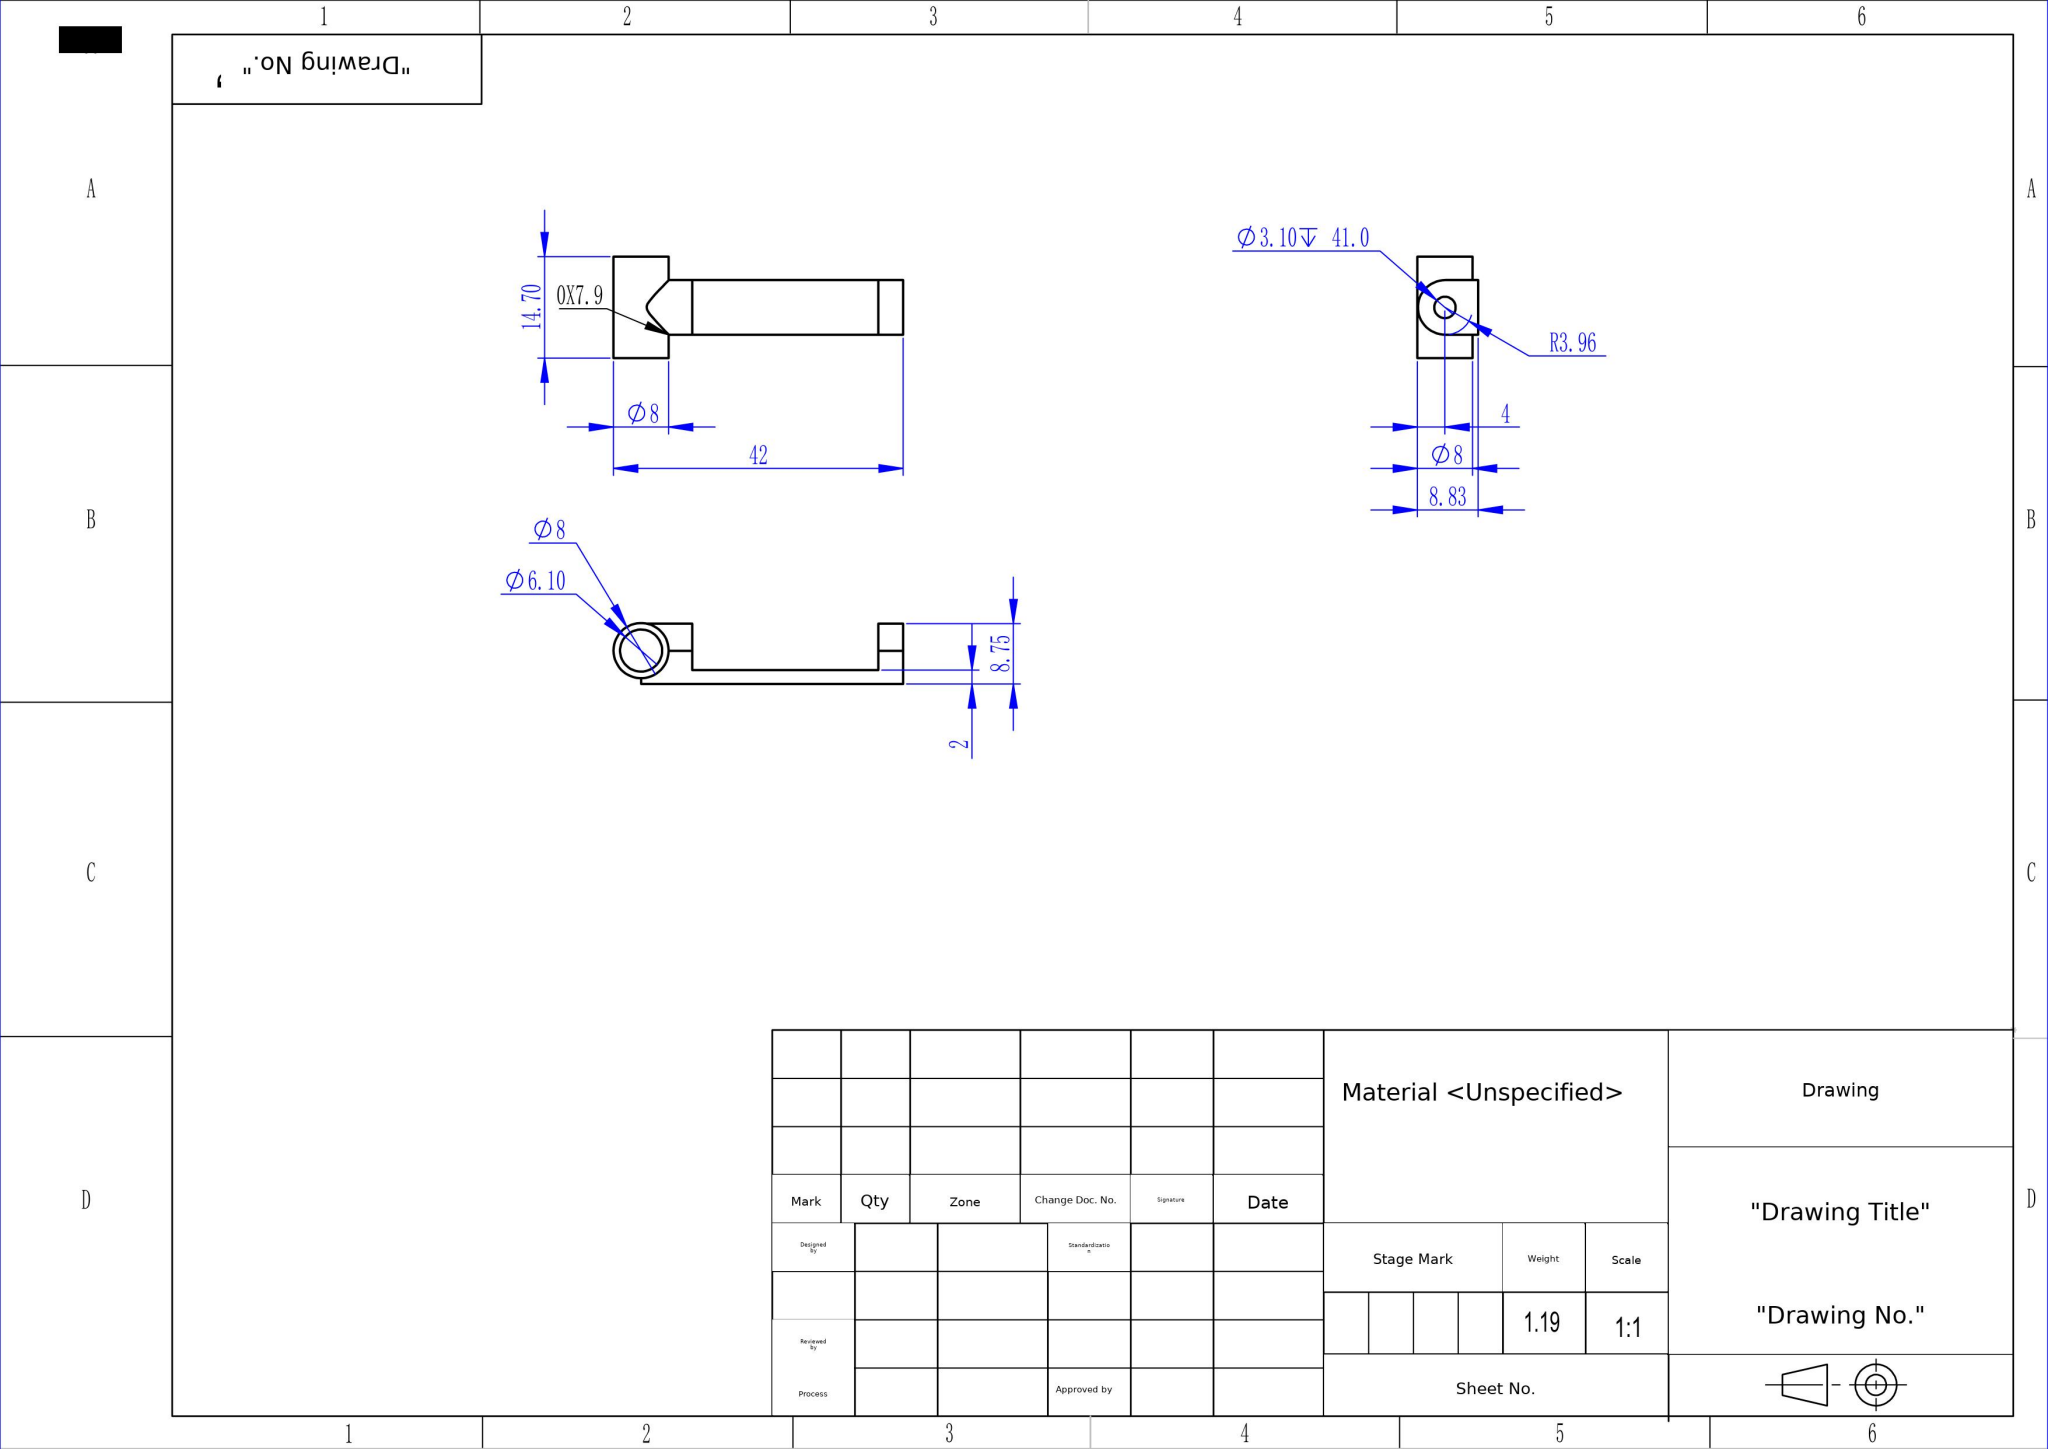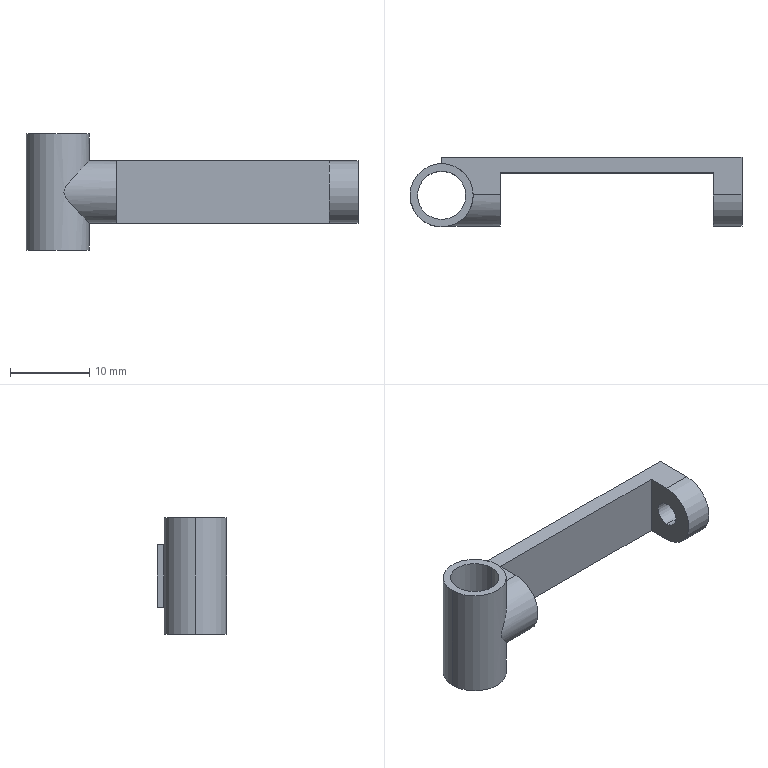Part | SolidWorks | mm | 1 solid | 21 faces | box 42 x 8.83 x 14.7 mm | volume 1194 mm3 | plane 11 | cylinder 10 | commonest cylinder face diameters 3.1 x4 6.1 x2 8 x2 7.923 x2
build123d program:
from build123d import *

# Parameters (mm, degrees)
SKETCH1_R           = 4
SKETCH1_R_2         = 3.05
BOSS_EXTRUDE1_DEPTH = 14.7
BOSS_EXTRUDE2_DEPTH = 38
CUT_EXTRUDE1_START  = -2
SKETCH3_W           = 26.966
SKETCH3_H           = 7.923
CUT_EXTRUDE1_DEPTH  = 30
CUT_EXTRUDE2_START  = -3
SKETCH4_R           = 1.55
CUT_EXTRUDE2_DEPTH  = 41
SKETCH5_R           = 3.05
CUT_EXTRUDE3_DEPTH  = 17


with BuildPart() as part:
    # Sketch1 → Boss-Extrude1 (new body)
    with BuildSketch(Plane.XY):
        Circle(SKETCH1_R)
        Circle(SKETCH1_R_2, mode=Mode.SUBTRACT)
    extrude(amount=BOSS_EXTRUDE1_DEPTH)

    # Sketch2 → Boss-Extrude2 (add)
    with BuildSketch(Plane(origin=(0, 0, 0), x_dir=(0, 0, -1), z_dir=(1, 0, 0))):
        with BuildLine():
            Line((-3.389, 4.83), (-11.311, 4.83))
            Line((-11.311, 4.83), (-11.311, 0.04196))
            ThreePointArc((-11.311, 0.04196), (-7.35, -3.919), (-3.389, 0.04196))
            Line((-3.389, 0.04196), (-3.389, 4.83))
        make_face()
    extrude(amount=BOSS_EXTRUDE2_DEPTH)

    # Sketch3 → Cut-Extrude1 (cut)
    with BuildSketch(Plane(origin=(0, 4.83, 0), x_dir=(1, 0, 0), z_dir=(0, 1, 0)).offset(CUT_EXTRUDE1_START)):
        with Locations((20.909, -7.35)):
            Rectangle(SKETCH3_W, SKETCH3_H)
    extrude(amount=-CUT_EXTRUDE1_DEPTH, mode=Mode.SUBTRACT)

    # Sketch4 → Cut-Extrude2 (cut)
    with BuildSketch(Plane(origin=(7.426, 0, 0), x_dir=(0, 0, -1), z_dir=(1, 0, 0)).offset(CUT_EXTRUDE2_START)):
        with Locations(Location((-7.35, 0, 0), (0, 0, 180))):
            Circle(SKETCH4_R)
    extrude(amount=CUT_EXTRUDE2_DEPTH, mode=Mode.SUBTRACT)

    # Sketch5 → Cut-Extrude3 (cut)
    with BuildSketch(Plane(origin=(0, 0, 0), x_dir=(-1, 0, 0), z_dir=(0, 0, -1))):
        with Locations(Location((0, 0, 0), (0, 0, 180))):
            Circle(SKETCH5_R)
    extrude(amount=-CUT_EXTRUDE3_DEPTH, mode=Mode.SUBTRACT)


solid = part.part
STEP:
#1=CARTESIAN_POINT('',(38.,0.,5.8));
#2=VERTEX_POINT('',#1);
#3=CARTESIAN_POINT('',(38.,0.,8.9));
#4=VERTEX_POINT('',#3);
#5=CARTESIAN_POINT('',(38.,0.,7.35));
#6=DIRECTION('',(-1.,0.,0.));
#7=DIRECTION('',(0.,0.,-1.));
#8=AXIS2_PLACEMENT_3D('',#5,#6,#7);
#9=CIRCLE('',#8,1.55);
#10=EDGE_CURVE('',#2,#4,#9,.T.);
#11=ORIENTED_EDGE('',*,*,#10,.F.);
#12=CARTESIAN_POINT('',(34.392,0.,5.8));
#13=VERTEX_POINT('',#12);
#14=CARTESIAN_POINT('',(45.426,0.,5.8));
#15=DIRECTION('',(-1.,0.,0.));
#16=VECTOR('',#15,1000.);
#17=LINE('',#14,#16);
#18=EDGE_CURVE('',#2,#13,#17,.T.);
#19=ORIENTED_EDGE('',*,*,#18,.T.);
#20=CARTESIAN_POINT('',(34.392,0.,8.9));
#21=VERTEX_POINT('',#20);
#22=CARTESIAN_POINT('',(34.392,0.,7.35));
#23=DIRECTION('',(-1.,0.,0.));
#24=DIRECTION('',(0.,0.,-1.));
#25=AXIS2_PLACEMENT_3D('',#22,#23,#24);
#26=CIRCLE('',#25,1.55);
#27=EDGE_CURVE('',#13,#21,#26,.T.);
#28=ORIENTED_EDGE('',*,*,#27,.T.);
#29=CARTESIAN_POINT('',(45.426,0.,8.9));
#30=DIRECTION('',(-1.,0.,0.));
#31=VECTOR('',#30,1000.);
#32=LINE('',#29,#31);
#33=EDGE_CURVE('',#4,#21,#32,.T.);
#34=ORIENTED_EDGE('',*,*,#33,.F.);
#35=EDGE_LOOP('',(#11,#19,#28,#34));
#36=FACE_OUTER_BOUND('',#35,.T.);
#37=CARTESIAN_POINT('',(45.426,0.,7.35));
#38=DIRECTION('',(-1.,0.,0.));
#39=DIRECTION('',(0.,0.,1.));
#40=AXIS2_PLACEMENT_3D('',#37,#38,#39);
#41=CYLINDRICAL_SURFACE('',#40,1.55);
#42=ADVANCED_FACE('',(#36),#41,.F.);
#43=CARTESIAN_POINT('',(7.426,0.,8.9));
#44=VERTEX_POINT('',#43);
#45=CARTESIAN_POINT('',(7.426,0.,5.8));
#46=VERTEX_POINT('',#45);
#47=CARTESIAN_POINT('',(7.426,0.,7.35));
#48=DIRECTION('',(1.,0.,0.));
#49=DIRECTION('',(0.,0.,1.));
#50=AXIS2_PLACEMENT_3D('',#47,#48,#49);
#51=CIRCLE('',#50,1.55);
#52=EDGE_CURVE('',#44,#46,#51,.T.);
#53=ORIENTED_EDGE('',*,*,#52,.T.);
#54=CARTESIAN_POINT('',(4.426,0.,5.8));
#55=VERTEX_POINT('',#54);
#56=CARTESIAN_POINT('',(45.426,0.,5.8));
#57=DIRECTION('',(-1.,0.,0.));
#58=VECTOR('',#57,1000.);
#59=LINE('',#56,#58);
#60=EDGE_CURVE('',#46,#55,#59,.T.);
#61=ORIENTED_EDGE('',*,*,#60,.T.);
#62=CARTESIAN_POINT('',(4.426,0.,8.9));
#63=VERTEX_POINT('',#62);
#64=CARTESIAN_POINT('',(4.426,0.,7.35));
#65=DIRECTION('',(1.,0.,0.));
#66=DIRECTION('',(0.,0.,-1.));
#67=AXIS2_PLACEMENT_3D('',#64,#65,#66);
#68=CIRCLE('',#67,1.55);
#69=EDGE_CURVE('',#63,#55,#68,.T.);
#70=ORIENTED_EDGE('',*,*,#69,.F.);
#71=CARTESIAN_POINT('',(45.426,0.,8.9));
#72=DIRECTION('',(-1.,0.,0.));
#73=VECTOR('',#72,1000.);
#74=LINE('',#71,#73);
#75=EDGE_CURVE('',#44,#63,#74,.T.);
#76=ORIENTED_EDGE('',*,*,#75,.F.);
#77=EDGE_LOOP('',(#53,#61,#70,#76));
#78=FACE_OUTER_BOUND('',#77,.T.);
#79=CARTESIAN_POINT('',(45.426,0.,7.35));
#80=DIRECTION('',(-1.,0.,0.));
#81=DIRECTION('',(0.,0.,1.));
#82=AXIS2_PLACEMENT_3D('',#79,#80,#81);
#83=CYLINDRICAL_SURFACE('',#82,1.55);
#84=ADVANCED_FACE('',(#78),#83,.F.);
#85=CARTESIAN_POINT('',(-3.05,0.,14.7));
#86=VERTEX_POINT('',#85);
#87=CARTESIAN_POINT('',(3.05,0.,14.7));
#88=VERTEX_POINT('',#87);
#89=CARTESIAN_POINT('',(0.,0.,14.7));
#90=DIRECTION('',(0.,0.,1.));
#91=DIRECTION('',(1.,0.,0.));
#92=AXIS2_PLACEMENT_3D('',#89,#90,#91);
#93=CIRCLE('',#92,3.05);
#94=EDGE_CURVE('',#86,#88,#93,.T.);
#95=ORIENTED_EDGE('',*,*,#94,.T.);
#96=CARTESIAN_POINT('',(3.05,0.,0.));
#97=VERTEX_POINT('',#96);
#98=CARTESIAN_POINT('',(3.05,0.,14.7));
#99=DIRECTION('',(0.,0.,-1.));
#100=VECTOR('',#99,1000.);
#101=LINE('',#98,#100);
#102=EDGE_CURVE('',#88,#97,#101,.T.);
#103=ORIENTED_EDGE('',*,*,#102,.T.);
#104=CARTESIAN_POINT('',(-3.05,0.,0.));
#105=VERTEX_POINT('',#104);
#106=CARTESIAN_POINT('',(0.,0.,0.));
#107=DIRECTION('',(0.,0.,1.));
#108=DIRECTION('',(1.,0.,0.));
#109=AXIS2_PLACEMENT_3D('',#106,#107,#108);
#110=CIRCLE('',#109,3.05);
#111=EDGE_CURVE('',#105,#97,#110,.T.);
#112=ORIENTED_EDGE('',*,*,#111,.F.);
#113=CARTESIAN_POINT('',(-3.05,0.,14.7));
#114=DIRECTION('',(0.,0.,-1.));
#115=VECTOR('',#114,1000.);
#116=LINE('',#113,#115);
#117=EDGE_CURVE('',#86,#105,#116,.T.);
#118=ORIENTED_EDGE('',*,*,#117,.F.);
#119=EDGE_LOOP('',(#95,#103,#112,#118));
#120=FACE_OUTER_BOUND('',#119,.T.);
#121=CARTESIAN_POINT('',(0.,0.,14.7));
#122=DIRECTION('',(0.,0.,-1.));
#123=DIRECTION('',(-1.,0.,0.));
#124=AXIS2_PLACEMENT_3D('',#121,#122,#123);
#125=CYLINDRICAL_SURFACE('',#124,3.05);
#126=ADVANCED_FACE('',(#120),#125,.F.);
#127=CARTESIAN_POINT('',(4.,0.,14.7));
#128=VERTEX_POINT('',#127);
#129=CARTESIAN_POINT('',(-4.,0.,14.7));
#130=VERTEX_POINT('',#129);
#131=CARTESIAN_POINT('',(0.,0.,14.7));
#132=DIRECTION('',(0.,0.,1.));
#133=DIRECTION('',(1.,0.,0.));
#134=AXIS2_PLACEMENT_3D('',#131,#132,#133);
#135=CIRCLE('',#134,4.);
#136=EDGE_CURVE('',#128,#130,#135,.T.);
#137=ORIENTED_EDGE('',*,*,#136,.F.);
#138=CARTESIAN_POINT('',(4.,0.,11.311));
#139=VERTEX_POINT('',#138);
#140=CARTESIAN_POINT('',(4.,0.,14.7));
#141=DIRECTION('',(0.,0.,-1.));
#142=VECTOR('',#141,1000.);
#143=LINE('',#140,#142);
#144=EDGE_CURVE('',#128,#139,#143,.T.);
#145=ORIENTED_EDGE('',*,*,#144,.T.);
#146=CARTESIAN_POINT('',(4.,0.04196,11.311));
#147=VERTEX_POINT('',#146);
#148=CARTESIAN_POINT('',(4.,0.04196,11.311));
#149=CARTESIAN_POINT('',(4.,0.03497,11.311));
#150=CARTESIAN_POINT('',(4.,0.02098,11.311));
#151=CARTESIAN_POINT('',(4.,0.006991,11.311));
#152=CARTESIAN_POINT('',(4.,0.,11.311));
#153=B_SPLINE_CURVE_WITH_KNOTS('',3,(#148,#149,#150,#151,#152),.UNSPECIFIED.,.F.,.F.,(4,1,4),(0.01481,0.01483,0.01485),.UNSPECIFIED.);
#154=EDGE_CURVE('',#147,#139,#153,.T.);
#155=ORIENTED_EDGE('',*,*,#154,.F.);
#156=CARTESIAN_POINT('',(0.,4.,11.311));
#157=VERTEX_POINT('',#156);
#158=CARTESIAN_POINT('',(0.,0.,11.311));
#159=DIRECTION('',(0.,-0.,-1.));
#160=DIRECTION('',(0.,1.,-0.));
#161=AXIS2_PLACEMENT_3D('',#158,#159,#160);
#162=CIRCLE('',#161,4.);
#163=EDGE_CURVE('',#157,#147,#162,.T.);
#164=ORIENTED_EDGE('',*,*,#163,.F.);
#165=CARTESIAN_POINT('',(0.,4.,3.389));
#166=VERTEX_POINT('',#165);
#167=CARTESIAN_POINT('',(0.,4.,14.7));
#168=DIRECTION('',(0.,0.,1.));
#169=VECTOR('',#168,1000.);
#170=LINE('',#167,#169);
#171=EDGE_CURVE('',#166,#157,#170,.T.);
#172=ORIENTED_EDGE('',*,*,#171,.F.);
#173=CARTESIAN_POINT('',(4.,0.04196,3.389));
#174=VERTEX_POINT('',#173);
#175=CARTESIAN_POINT('',(0.,0.,3.389));
#176=DIRECTION('',(0.,0.,-1.));
#177=DIRECTION('',(0.,1.,0.));
#178=AXIS2_PLACEMENT_3D('',#175,#176,#177);
#179=CIRCLE('',#178,4.);
#180=EDGE_CURVE('',#166,#174,#179,.T.);
#181=ORIENTED_EDGE('',*,*,#180,.T.);
#182=CARTESIAN_POINT('',(4.,0.,3.389));
#183=VERTEX_POINT('',#182);
#184=CARTESIAN_POINT('',(4.,0.,3.389));
#185=CARTESIAN_POINT('',(4.,0.006996,3.389));
#186=CARTESIAN_POINT('',(4.,0.02099,3.389));
#187=CARTESIAN_POINT('',(4.,0.03497,3.389));
#188=CARTESIAN_POINT('',(4.,0.04196,3.389));
#189=B_SPLINE_CURVE_WITH_KNOTS('',3,(#184,#185,#186,#187,#188),.UNSPECIFIED.,.F.,.F.,(4,1,4),(0.02866,0.02868,0.0287),.UNSPECIFIED.);
#190=EDGE_CURVE('',#183,#174,#189,.T.);
#191=ORIENTED_EDGE('',*,*,#190,.F.);
#192=CARTESIAN_POINT('',(4.,0.,0.));
#193=VERTEX_POINT('',#192);
#194=CARTESIAN_POINT('',(4.,0.,14.7));
#195=DIRECTION('',(0.,0.,-1.));
#196=VECTOR('',#195,1000.);
#197=LINE('',#194,#196);
#198=EDGE_CURVE('',#183,#193,#197,.T.);
#199=ORIENTED_EDGE('',*,*,#198,.T.);
#200=CARTESIAN_POINT('',(-4.,0.,0.));
#201=VERTEX_POINT('',#200);
#202=CARTESIAN_POINT('',(0.,0.,0.));
#203=DIRECTION('',(0.,0.,1.));
#204=DIRECTION('',(1.,0.,0.));
#205=AXIS2_PLACEMENT_3D('',#202,#203,#204);
#206=CIRCLE('',#205,4.);
#207=EDGE_CURVE('',#193,#201,#206,.T.);
#208=ORIENTED_EDGE('',*,*,#207,.T.);
#209=CARTESIAN_POINT('',(-4.,0.,14.7));
#210=DIRECTION('',(0.,0.,-1.));
#211=VECTOR('',#210,1000.);
#212=LINE('',#209,#211);
#213=EDGE_CURVE('',#130,#201,#212,.T.);
#214=ORIENTED_EDGE('',*,*,#213,.F.);
#215=EDGE_LOOP('',(#137,#145,#155,#164,#172,#181,#191,#199,#208,#214));
#216=FACE_OUTER_BOUND('',#215,.T.);
#217=CARTESIAN_POINT('',(0.,0.,14.7));
#218=DIRECTION('',(0.,0.,-1.));
#219=DIRECTION('',(-1.,0.,0.));
#220=AXIS2_PLACEMENT_3D('',#217,#218,#219);
#221=CYLINDRICAL_SURFACE('',#220,4.);
#222=ADVANCED_FACE('',(#216),#221,.T.);
#223=CARTESIAN_POINT('',(38.,0.04196,11.311));
#224=VERTEX_POINT('',#223);
#225=CARTESIAN_POINT('',(34.392,0.04196,11.311));
#226=VERTEX_POINT('',#225);
#227=CARTESIAN_POINT('',(38.,0.04196,11.311));
#228=DIRECTION('',(-1.,0.,0.));
#229=VECTOR('',#228,1000.);
#230=LINE('',#227,#229);
#231=EDGE_CURVE('',#224,#226,#230,.T.);
#232=ORIENTED_EDGE('',*,*,#231,.T.);
#233=CARTESIAN_POINT('',(34.392,0.04196,3.389));
#234=VERTEX_POINT('',#233);
#235=CARTESIAN_POINT('',(34.392,0.04196,7.35));
#236=DIRECTION('',(1.,0.,0.));
#237=DIRECTION('',(0.,0.,-1.));
#238=AXIS2_PLACEMENT_3D('',#235,#236,#237);
#239=CIRCLE('',#238,3.961);
#240=EDGE_CURVE('',#226,#234,#239,.T.);
#241=ORIENTED_EDGE('',*,*,#240,.T.);
#242=CARTESIAN_POINT('',(38.,0.04196,3.389));
#243=VERTEX_POINT('',#242);
#244=CARTESIAN_POINT('',(38.,0.04196,3.389));
#245=DIRECTION('',(-1.,0.,0.));
#246=VECTOR('',#245,1000.);
#247=LINE('',#244,#246);
#248=EDGE_CURVE('',#243,#234,#247,.T.);
#249=ORIENTED_EDGE('',*,*,#248,.F.);
#250=CARTESIAN_POINT('',(38.,0.04196,7.35));
#251=DIRECTION('',(1.,0.,0.));
#252=DIRECTION('',(0.,0.,-1.));
#253=AXIS2_PLACEMENT_3D('',#250,#251,#252);
#254=CIRCLE('',#253,3.961);
#255=EDGE_CURVE('',#224,#243,#254,.T.);
#256=ORIENTED_EDGE('',*,*,#255,.F.);
#257=EDGE_LOOP('',(#232,#241,#249,#256));
#258=FACE_OUTER_BOUND('',#257,.T.);
#259=CARTESIAN_POINT('',(38.,0.04196,7.35));
#260=DIRECTION('',(-1.,0.,0.));
#261=DIRECTION('',(0.,0.,1.));
#262=AXIS2_PLACEMENT_3D('',#259,#260,#261);
#263=CYLINDRICAL_SURFACE('',#262,3.961);
#264=ADVANCED_FACE('',(#258),#263,.T.);
#265=ORIENTED_EDGE('',*,*,#144,.F.);
#266=CARTESIAN_POINT('',(0.,0.,14.7));
#267=DIRECTION('',(0.,0.,1.));
#268=DIRECTION('',(1.,0.,0.));
#269=AXIS2_PLACEMENT_3D('',#266,#267,#268);
#270=CIRCLE('',#269,4.);
#271=EDGE_CURVE('',#130,#128,#270,.T.);
#272=ORIENTED_EDGE('',*,*,#271,.F.);
#273=ORIENTED_EDGE('',*,*,#213,.T.);
#274=CARTESIAN_POINT('',(0.,0.,0.));
#275=DIRECTION('',(0.,0.,1.));
#276=DIRECTION('',(1.,0.,0.));
#277=AXIS2_PLACEMENT_3D('',#274,#275,#276);
#278=CIRCLE('',#277,4.);
#279=EDGE_CURVE('',#201,#193,#278,.T.);
#280=ORIENTED_EDGE('',*,*,#279,.T.);
#281=ORIENTED_EDGE('',*,*,#198,.F.);
#282=CARTESIAN_POINT('',(4.,0.,11.311));
#283=CARTESIAN_POINT('',(4.,-0.147,11.31));
#284=CARTESIAN_POINT('',(3.992,-0.2933,11.3));
#285=CARTESIAN_POINT('',(3.96,-0.5848,11.264));
#286=CARTESIAN_POINT('',(3.935,-0.7306,11.238));
#287=CARTESIAN_POINT('',(3.873,-1.012,11.171));
#288=CARTESIAN_POINT('',(3.834,-1.148,11.131));
#289=CARTESIAN_POINT('',(3.745,-1.413,11.037));
#290=CARTESIAN_POINT('',(3.693,-1.543,10.983));
#291=CARTESIAN_POINT('',(3.523,-1.913,10.806));
#292=CARTESIAN_POINT('',(3.391,-2.136,10.669));
#293=CARTESIAN_POINT('',(3.097,-2.544,10.361));
#294=CARTESIAN_POINT('',(2.934,-2.728,10.192));
#295=CARTESIAN_POINT('',(2.598,-3.051,9.837));
#296=CARTESIAN_POINT('',(2.421,-3.192,9.65));
#297=CARTESIAN_POINT('',(2.057,-3.437,9.258));
#298=CARTESIAN_POINT('',(1.869,-3.542,9.052));
#299=CARTESIAN_POINT('',(1.5,-3.714,8.63));
#300=CARTESIAN_POINT('',(1.315,-3.782,8.413));
#301=CARTESIAN_POINT('',(1.062,-3.857,8.059));
#302=CARTESIAN_POINT('',(0.9816,-3.878,7.935));
#303=CARTESIAN_POINT('',(0.8837,-3.901,7.734));
#304=CARTESIAN_POINT('',(0.8556,-3.907,7.665));
#305=CARTESIAN_POINT('',(0.8141,-3.916,7.522));
#306=CARTESIAN_POINT('',(0.8013,-3.919,7.447));
#307=CARTESIAN_POINT('',(0.7952,-3.92,7.223));
#308=CARTESIAN_POINT('',(0.8363,-3.912,7.074));
#309=CARTESIAN_POINT('',(0.9595,-3.884,6.802));
#310=CARTESIAN_POINT('',(1.038,-3.864,6.678));
#311=CARTESIAN_POINT('',(1.289,-3.791,6.318));
#312=CARTESIAN_POINT('',(1.478,-3.723,6.096));
#313=CARTESIAN_POINT('',(1.85,-3.552,5.669));
#314=CARTESIAN_POINT('',(2.037,-3.45,5.464));
#315=CARTESIAN_POINT('',(2.404,-3.204,5.068));
#316=CARTESIAN_POINT('',(2.585,-3.062,4.877));
#317=CARTESIAN_POINT('',(2.925,-2.739,4.518));
#318=CARTESIAN_POINT('',(3.086,-2.558,4.35));
#319=CARTESIAN_POINT('',(3.384,-2.147,4.038));
#320=CARTESIAN_POINT('',(3.519,-1.921,3.898));
#321=CARTESIAN_POINT('',(3.746,-1.428,3.662));
#322=CARTESIAN_POINT('',(3.84,-1.157,3.564));
#323=CARTESIAN_POINT('',(3.934,-0.7358,3.463));
#324=CARTESIAN_POINT('',(3.959,-0.592,3.437));
#325=CARTESIAN_POINT('',(3.992,-0.2975,3.4));
#326=CARTESIAN_POINT('',(4.,-0.1479,3.39));
#327=CARTESIAN_POINT('',(4.,0.,3.389));
#328=B_SPLINE_CURVE_WITH_KNOTS('',3,(#282,#283,#284,#285,#286,#287,#288,#289,#290,#291,#292,#293,#294,#295,#296,#297,#298,#299,#300,#301,#302,#303,#304,#305,#306,#307,#308,#309,#310,#311,#312,#313,#314,#315,#316,#317,#318,#319,#320,#321,#322,#323,#324,#325,#326,#327),.UNSPECIFIED.,.F.,.F.,(4,2,2,2,2,2,2,2,2,2,2,2,2,2,2,2,2,2,2,2,2,2,4),(0.01485,0.01528,0.01571,0.01614,0.01657,0.01744,0.0183,0.01916,0.02003,0.02089,0.02132,0.02154,0.02175,0.02219,0.02262,0.02348,0.02434,0.02521,0.02607,0.02693,0.0278,0.02823,0.02866),.UNSPECIFIED.);
#329=EDGE_CURVE('',#139,#183,#328,.T.);
#330=ORIENTED_EDGE('',*,*,#329,.F.);
#331=EDGE_LOOP('',(#265,#272,#273,#280,#281,#330));
#332=FACE_OUTER_BOUND('',#331,.T.);
#333=CARTESIAN_POINT('',(0.,0.,14.7));
#334=DIRECTION('',(0.,0.,-1.));
#335=DIRECTION('',(-1.,0.,0.));
#336=AXIS2_PLACEMENT_3D('',#333,#334,#335);
#337=CYLINDRICAL_SURFACE('',#336,4.);
#338=ADVANCED_FACE('',(#332),#337,.T.);
#339=ORIENTED_EDGE('',*,*,#102,.F.);
#340=CARTESIAN_POINT('',(0.,0.,14.7));
#341=DIRECTION('',(0.,0.,1.));
#342=DIRECTION('',(1.,0.,0.));
#343=AXIS2_PLACEMENT_3D('',#340,#341,#342);
#344=CIRCLE('',#343,3.05);
#345=EDGE_CURVE('',#88,#86,#344,.T.);
#346=ORIENTED_EDGE('',*,*,#345,.T.);
#347=ORIENTED_EDGE('',*,*,#117,.T.);
#348=CARTESIAN_POINT('',(0.,0.,0.));
#349=DIRECTION('',(0.,0.,1.));
#350=DIRECTION('',(1.,0.,0.));
#351=AXIS2_PLACEMENT_3D('',#348,#349,#350);
#352=CIRCLE('',#351,3.05);
#353=EDGE_CURVE('',#97,#105,#352,.T.);
#354=ORIENTED_EDGE('',*,*,#353,.F.);
#355=EDGE_LOOP('',(#339,#346,#347,#354));
#356=FACE_OUTER_BOUND('',#355,.T.);
#357=CARTESIAN_POINT('',(0.,0.,14.7));
#358=DIRECTION('',(0.,0.,-1.));
#359=DIRECTION('',(-1.,0.,0.));
#360=AXIS2_PLACEMENT_3D('',#357,#358,#359);
#361=CYLINDRICAL_SURFACE('',#360,3.05);
#362=ADVANCED_FACE('',(#356),#361,.F.);
#363=ORIENTED_EDGE('',*,*,#271,.T.);
#364=ORIENTED_EDGE('',*,*,#136,.T.);
#365=EDGE_LOOP('',(#363,#364));
#366=FACE_OUTER_BOUND('',#365,.T.);
#367=ORIENTED_EDGE('',*,*,#94,.F.);
#368=ORIENTED_EDGE('',*,*,#345,.F.);
#369=EDGE_LOOP('',(#367,#368));
#370=FACE_BOUND('',#369,.T.);
#371=CARTESIAN_POINT('',(0.,0.,14.7));
#372=DIRECTION('',(0.,0.,1.));
#373=DIRECTION('',(1.,0.,0.));
#374=AXIS2_PLACEMENT_3D('',#371,#372,#373);
#375=PLANE('',#374);
#376=ADVANCED_FACE('',(#366,#370),#375,.T.);
#377=ORIENTED_EDGE('',*,*,#279,.F.);
#378=ORIENTED_EDGE('',*,*,#207,.F.);
#379=EDGE_LOOP('',(#377,#378));
#380=FACE_OUTER_BOUND('',#379,.T.);
#381=ORIENTED_EDGE('',*,*,#111,.T.);
#382=ORIENTED_EDGE('',*,*,#353,.T.);
#383=EDGE_LOOP('',(#381,#382));
#384=FACE_BOUND('',#383,.T.);
#385=CARTESIAN_POINT('',(0.,0.,0.));
#386=DIRECTION('',(0.,0.,1.));
#387=DIRECTION('',(1.,0.,0.));
#388=AXIS2_PLACEMENT_3D('',#385,#386,#387);
#389=PLANE('',#388);
#390=ADVANCED_FACE('',(#380,#384),#389,.F.);
#391=CARTESIAN_POINT('',(7.426,0.04196,3.389));
#392=VERTEX_POINT('',#391);
#393=CARTESIAN_POINT('',(38.,0.04196,3.389));
#394=DIRECTION('',(-1.,0.,0.));
#395=VECTOR('',#394,1000.);
#396=LINE('',#393,#395);
#397=EDGE_CURVE('',#392,#174,#396,.T.);
#398=ORIENTED_EDGE('',*,*,#397,.F.);
#399=CARTESIAN_POINT('',(7.426,0.04196,11.311));
#400=VERTEX_POINT('',#399);
#401=CARTESIAN_POINT('',(7.426,0.04196,7.35));
#402=DIRECTION('',(-1.,0.,0.));
#403=DIRECTION('',(0.,0.,1.));
#404=AXIS2_PLACEMENT_3D('',#401,#402,#403);
#405=CIRCLE('',#404,3.961);
#406=EDGE_CURVE('',#392,#400,#405,.T.);
#407=ORIENTED_EDGE('',*,*,#406,.T.);
#408=CARTESIAN_POINT('',(38.,0.04196,11.311));
#409=DIRECTION('',(-1.,0.,0.));
#410=VECTOR('',#409,1000.);
#411=LINE('',#408,#410);
#412=EDGE_CURVE('',#400,#147,#411,.T.);
#413=ORIENTED_EDGE('',*,*,#412,.T.);
#414=ORIENTED_EDGE('',*,*,#154,.T.);
#415=ORIENTED_EDGE('',*,*,#329,.T.);
#416=ORIENTED_EDGE('',*,*,#190,.T.);
#417=EDGE_LOOP('',(#398,#407,#413,#414,#415,#416));
#418=FACE_OUTER_BOUND('',#417,.T.);
#419=CARTESIAN_POINT('',(38.,0.04196,7.35));
#420=DIRECTION('',(-1.,0.,0.));
#421=DIRECTION('',(0.,0.,1.));
#422=AXIS2_PLACEMENT_3D('',#419,#420,#421);
#423=CYLINDRICAL_SURFACE('',#422,3.961);
#424=ADVANCED_FACE('',(#418),#423,.T.);
#425=CARTESIAN_POINT('',(0.,4.83,3.389));
#426=VERTEX_POINT('',#425);
#427=CARTESIAN_POINT('',(0.,-0.,3.389));
#428=DIRECTION('',(0.,-1.,-0.));
#429=VECTOR('',#428,1000.);
#430=LINE('',#427,#429);
#431=EDGE_CURVE('',#426,#166,#430,.T.);
#432=ORIENTED_EDGE('',*,*,#431,.T.);
#433=ORIENTED_EDGE('',*,*,#171,.T.);
#434=CARTESIAN_POINT('',(0.,4.83,11.311));
#435=VERTEX_POINT('',#434);
#436=CARTESIAN_POINT('',(0.,0.,11.311));
#437=DIRECTION('',(0.,-1.,0.));
#438=VECTOR('',#437,1000.);
#439=LINE('',#436,#438);
#440=EDGE_CURVE('',#435,#157,#439,.T.);
#441=ORIENTED_EDGE('',*,*,#440,.F.);
#442=CARTESIAN_POINT('',(0.,4.83,0.));
#443=DIRECTION('',(0.,0.,1.));
#444=VECTOR('',#443,1000.);
#445=LINE('',#442,#444);
#446=EDGE_CURVE('',#426,#435,#445,.T.);
#447=ORIENTED_EDGE('',*,*,#446,.F.);
#448=EDGE_LOOP('',(#432,#433,#441,#447));
#449=FACE_OUTER_BOUND('',#448,.T.);
#450=CARTESIAN_POINT('',(0.,0.,0.));
#451=DIRECTION('',(1.,0.,0.));
#452=DIRECTION('',(0.,0.,-1.));
#453=AXIS2_PLACEMENT_3D('',#450,#451,#452);
#454=PLANE('',#453);
#455=ADVANCED_FACE('',(#449),#454,.F.);
#456=ORIENTED_EDGE('',*,*,#446,.T.);
#457=CARTESIAN_POINT('',(38.,4.83,11.311));
#458=VERTEX_POINT('',#457);
#459=CARTESIAN_POINT('',(38.,4.83,11.311));
#460=DIRECTION('',(-1.,0.,0.));
#461=VECTOR('',#460,1000.);
#462=LINE('',#459,#461);
#463=EDGE_CURVE('',#458,#435,#462,.T.);
#464=ORIENTED_EDGE('',*,*,#463,.F.);
#465=CARTESIAN_POINT('',(38.,4.83,3.389));
#466=VERTEX_POINT('',#465);
#467=CARTESIAN_POINT('',(38.,4.83,0.));
#468=DIRECTION('',(0.,0.,1.));
#469=VECTOR('',#468,1000.);
#470=LINE('',#467,#469);
#471=EDGE_CURVE('',#466,#458,#470,.T.);
#472=ORIENTED_EDGE('',*,*,#471,.F.);
#473=CARTESIAN_POINT('',(38.,4.83,3.389));
#474=DIRECTION('',(-1.,0.,0.));
#475=VECTOR('',#474,1000.);
#476=LINE('',#473,#475);
#477=EDGE_CURVE('',#466,#426,#476,.T.);
#478=ORIENTED_EDGE('',*,*,#477,.T.);
#479=EDGE_LOOP('',(#456,#464,#472,#478));
#480=FACE_OUTER_BOUND('',#479,.T.);
#481=CARTESIAN_POINT('',(38.,4.83,0.));
#482=DIRECTION('',(0.,-1.,0.));
#483=DIRECTION('',(0.,0.,-1.));
#484=AXIS2_PLACEMENT_3D('',#481,#482,#483);
#485=PLANE('',#484);
#486=ADVANCED_FACE('',(#480),#485,.F.);
#487=CARTESIAN_POINT('',(7.426,2.83,11.311));
#488=VERTEX_POINT('',#487);
#489=CARTESIAN_POINT('',(34.392,2.83,11.311));
#490=VERTEX_POINT('',#489);
#491=CARTESIAN_POINT('',(34.392,2.83,11.311));
#492=DIRECTION('',(1.,0.,-0.));
#493=VECTOR('',#492,1000.);
#494=LINE('',#491,#493);
#495=EDGE_CURVE('',#488,#490,#494,.T.);
#496=ORIENTED_EDGE('',*,*,#495,.T.);
#497=CARTESIAN_POINT('',(34.392,-27.17,11.311));
#498=DIRECTION('',(0.,1.,0.));
#499=VECTOR('',#498,1000.);
#500=LINE('',#497,#499);
#501=EDGE_CURVE('',#226,#490,#500,.T.);
#502=ORIENTED_EDGE('',*,*,#501,.F.);
#503=ORIENTED_EDGE('',*,*,#231,.F.);
#504=CARTESIAN_POINT('',(38.,0.,11.311));
#505=DIRECTION('',(0.,-1.,0.));
#506=VECTOR('',#505,1000.);
#507=LINE('',#504,#506);
#508=EDGE_CURVE('',#458,#224,#507,.T.);
#509=ORIENTED_EDGE('',*,*,#508,.F.);
#510=ORIENTED_EDGE('',*,*,#463,.T.);
#511=ORIENTED_EDGE('',*,*,#440,.T.);
#512=ORIENTED_EDGE('',*,*,#163,.T.);
#513=ORIENTED_EDGE('',*,*,#412,.F.);
#514=CARTESIAN_POINT('',(7.426,-27.17,11.311));
#515=DIRECTION('',(0.,1.,0.));
#516=VECTOR('',#515,1000.);
#517=LINE('',#514,#516);
#518=EDGE_CURVE('',#400,#488,#517,.T.);
#519=ORIENTED_EDGE('',*,*,#518,.T.);
#520=EDGE_LOOP('',(#496,#502,#503,#509,#510,#511,#512,#513,#519));
#521=FACE_OUTER_BOUND('',#520,.T.);
#522=CARTESIAN_POINT('',(38.,0.,11.311));
#523=DIRECTION('',(0.,-0.,-1.));
#524=DIRECTION('',(0.,1.,-0.));
#525=AXIS2_PLACEMENT_3D('',#522,#523,#524);
#526=PLANE('',#525);
#527=ADVANCED_FACE('',(#521),#526,.F.);
#528=CARTESIAN_POINT('',(34.392,2.83,3.389));
#529=VERTEX_POINT('',#528);
#530=CARTESIAN_POINT('',(34.392,-0.,3.389));
#531=DIRECTION('',(0.,-1.,-0.));
#532=VECTOR('',#531,1000.);
#533=LINE('',#530,#532);
#534=EDGE_CURVE('',#529,#234,#533,.T.);
#535=ORIENTED_EDGE('',*,*,#534,.F.);
#536=CARTESIAN_POINT('',(7.426,2.83,3.389));
#537=VERTEX_POINT('',#536);
#538=CARTESIAN_POINT('',(34.392,2.83,3.389));
#539=DIRECTION('',(-1.,0.,0.));
#540=VECTOR('',#539,1000.);
#541=LINE('',#538,#540);
#542=EDGE_CURVE('',#529,#537,#541,.T.);
#543=ORIENTED_EDGE('',*,*,#542,.T.);
#544=CARTESIAN_POINT('',(7.426,-0.,3.389));
#545=DIRECTION('',(0.,1.,0.));
#546=VECTOR('',#545,1000.);
#547=LINE('',#544,#546);
#548=EDGE_CURVE('',#392,#537,#547,.T.);
#549=ORIENTED_EDGE('',*,*,#548,.F.);
#550=ORIENTED_EDGE('',*,*,#397,.T.);
#551=ORIENTED_EDGE('',*,*,#180,.F.);
#552=ORIENTED_EDGE('',*,*,#431,.F.);
#553=ORIENTED_EDGE('',*,*,#477,.F.);
#554=CARTESIAN_POINT('',(38.,-0.,3.389));
#555=DIRECTION('',(0.,-1.,-0.));
#556=VECTOR('',#555,1000.);
#557=LINE('',#554,#556);
#558=EDGE_CURVE('',#466,#243,#557,.T.);
#559=ORIENTED_EDGE('',*,*,#558,.T.);
#560=ORIENTED_EDGE('',*,*,#248,.T.);
#561=EDGE_LOOP('',(#535,#543,#549,#550,#551,#552,#553,#559,#560));
#562=FACE_OUTER_BOUND('',#561,.T.);
#563=CARTESIAN_POINT('',(38.,-0.,3.389));
#564=DIRECTION('',(0.,0.,-1.));
#565=DIRECTION('',(0.,1.,0.));
#566=AXIS2_PLACEMENT_3D('',#563,#564,#565);
#567=PLANE('',#566);
#568=ADVANCED_FACE('',(#562),#567,.T.);
#569=CARTESIAN_POINT('',(38.,0.,7.35));
#570=DIRECTION('',(-1.,0.,0.));
#571=DIRECTION('',(0.,0.,-1.));
#572=AXIS2_PLACEMENT_3D('',#569,#570,#571);
#573=CIRCLE('',#572,1.55);
#574=EDGE_CURVE('',#4,#2,#573,.T.);
#575=ORIENTED_EDGE('',*,*,#574,.T.);
#576=ORIENTED_EDGE('',*,*,#10,.T.);
#577=EDGE_LOOP('',(#575,#576));
#578=FACE_BOUND('',#577,.T.);
#579=ORIENTED_EDGE('',*,*,#471,.T.);
#580=ORIENTED_EDGE('',*,*,#508,.T.);
#581=ORIENTED_EDGE('',*,*,#255,.T.);
#582=ORIENTED_EDGE('',*,*,#558,.F.);
#583=EDGE_LOOP('',(#579,#580,#581,#582));
#584=FACE_OUTER_BOUND('',#583,.T.);
#585=CARTESIAN_POINT('',(38.,0.,0.));
#586=DIRECTION('',(1.,0.,0.));
#587=DIRECTION('',(0.,0.,-1.));
#588=AXIS2_PLACEMENT_3D('',#585,#586,#587);
#589=PLANE('',#588);
#590=ADVANCED_FACE('',(#578,#584),#589,.T.);
#591=CARTESIAN_POINT('',(34.392,0.,7.35));
#592=DIRECTION('',(-1.,0.,0.));
#593=DIRECTION('',(0.,0.,-1.));
#594=AXIS2_PLACEMENT_3D('',#591,#592,#593);
#595=CIRCLE('',#594,1.55);
#596=EDGE_CURVE('',#21,#13,#595,.T.);
#597=ORIENTED_EDGE('',*,*,#596,.F.);
#598=ORIENTED_EDGE('',*,*,#27,.F.);
#599=EDGE_LOOP('',(#597,#598));
#600=FACE_BOUND('',#599,.T.);
#601=ORIENTED_EDGE('',*,*,#501,.T.);
#602=CARTESIAN_POINT('',(34.392,2.83,3.389));
#603=DIRECTION('',(0.,0.,-1.));
#604=VECTOR('',#603,1000.);
#605=LINE('',#602,#604);
#606=EDGE_CURVE('',#490,#529,#605,.T.);
#607=ORIENTED_EDGE('',*,*,#606,.T.);
#608=ORIENTED_EDGE('',*,*,#534,.T.);
#609=ORIENTED_EDGE('',*,*,#240,.F.);
#610=EDGE_LOOP('',(#601,#607,#608,#609));
#611=FACE_OUTER_BOUND('',#610,.T.);
#612=CARTESIAN_POINT('',(34.392,-27.17,3.389));
#613=DIRECTION('',(1.,0.,0.));
#614=DIRECTION('',(0.,0.,-1.));
#615=AXIS2_PLACEMENT_3D('',#612,#613,#614);
#616=PLANE('',#615);
#617=ADVANCED_FACE('',(#600,#611),#616,.F.);
#618=ORIENTED_EDGE('',*,*,#52,.F.);
#619=CARTESIAN_POINT('',(7.426,0.,7.35));
#620=DIRECTION('',(1.,0.,0.));
#621=DIRECTION('',(0.,0.,1.));
#622=AXIS2_PLACEMENT_3D('',#619,#620,#621);
#623=CIRCLE('',#622,1.55);
#624=EDGE_CURVE('',#46,#44,#623,.T.);
#625=ORIENTED_EDGE('',*,*,#624,.F.);
#626=EDGE_LOOP('',(#618,#625));
#627=FACE_BOUND('',#626,.T.);
#628=ORIENTED_EDGE('',*,*,#548,.T.);
#629=CARTESIAN_POINT('',(7.426,2.83,3.389));
#630=DIRECTION('',(0.,0.,1.));
#631=VECTOR('',#630,1000.);
#632=LINE('',#629,#631);
#633=EDGE_CURVE('',#537,#488,#632,.T.);
#634=ORIENTED_EDGE('',*,*,#633,.T.);
#635=ORIENTED_EDGE('',*,*,#518,.F.);
#636=ORIENTED_EDGE('',*,*,#406,.F.);
#637=EDGE_LOOP('',(#628,#634,#635,#636));
#638=FACE_OUTER_BOUND('',#637,.T.);
#639=CARTESIAN_POINT('',(7.426,-27.17,3.389));
#640=DIRECTION('',(-1.,0.,0.));
#641=DIRECTION('',(0.,0.,1.));
#642=AXIS2_PLACEMENT_3D('',#639,#640,#641);
#643=PLANE('',#642);
#644=ADVANCED_FACE('',(#627,#638),#643,.F.);
#645=ORIENTED_EDGE('',*,*,#606,.F.);
#646=ORIENTED_EDGE('',*,*,#495,.F.);
#647=ORIENTED_EDGE('',*,*,#633,.F.);
#648=ORIENTED_EDGE('',*,*,#542,.F.);
#649=EDGE_LOOP('',(#645,#646,#647,#648));
#650=FACE_OUTER_BOUND('',#649,.T.);
#651=CARTESIAN_POINT('',(0.,2.83,0.));
#652=DIRECTION('',(0.,-1.,0.));
#653=DIRECTION('',(0.,0.,-1.));
#654=AXIS2_PLACEMENT_3D('',#651,#652,#653);
#655=PLANE('',#654);
#656=ADVANCED_FACE('',(#650),#655,.T.);
#657=ORIENTED_EDGE('',*,*,#69,.T.);
#658=CARTESIAN_POINT('',(4.426,0.,7.35));
#659=DIRECTION('',(1.,0.,0.));
#660=DIRECTION('',(0.,0.,-1.));
#661=AXIS2_PLACEMENT_3D('',#658,#659,#660);
#662=CIRCLE('',#661,1.55);
#663=EDGE_CURVE('',#55,#63,#662,.T.);
#664=ORIENTED_EDGE('',*,*,#663,.T.);
#665=EDGE_LOOP('',(#657,#664));
#666=FACE_OUTER_BOUND('',#665,.T.);
#667=CARTESIAN_POINT('',(4.426,0.,7.35));
#668=DIRECTION('',(1.,0.,0.));
#669=DIRECTION('',(0.,0.,-1.));
#670=AXIS2_PLACEMENT_3D('',#667,#668,#669);
#671=PLANE('',#670);
#672=ADVANCED_FACE('',(#666),#671,.T.);
#673=ORIENTED_EDGE('',*,*,#60,.F.);
#674=ORIENTED_EDGE('',*,*,#624,.T.);
#675=ORIENTED_EDGE('',*,*,#75,.T.);
#676=ORIENTED_EDGE('',*,*,#663,.F.);
#677=EDGE_LOOP('',(#673,#674,#675,#676));
#678=FACE_OUTER_BOUND('',#677,.T.);
#679=CARTESIAN_POINT('',(45.426,0.,7.35));
#680=DIRECTION('',(-1.,0.,0.));
#681=DIRECTION('',(0.,0.,1.));
#682=AXIS2_PLACEMENT_3D('',#679,#680,#681);
#683=CYLINDRICAL_SURFACE('',#682,1.55);
#684=ADVANCED_FACE('',(#678),#683,.F.);
#685=ORIENTED_EDGE('',*,*,#18,.F.);
#686=ORIENTED_EDGE('',*,*,#574,.F.);
#687=ORIENTED_EDGE('',*,*,#33,.T.);
#688=ORIENTED_EDGE('',*,*,#596,.T.);
#689=EDGE_LOOP('',(#685,#686,#687,#688));
#690=FACE_OUTER_BOUND('',#689,.T.);
#691=CARTESIAN_POINT('',(45.426,0.,7.35));
#692=DIRECTION('',(-1.,0.,0.));
#693=DIRECTION('',(0.,0.,1.));
#694=AXIS2_PLACEMENT_3D('',#691,#692,#693);
#695=CYLINDRICAL_SURFACE('',#694,1.55);
#696=ADVANCED_FACE('',(#690),#695,.F.);
#697=CLOSED_SHELL('',(#42,#84,#126,#222,#264,#338,#362,#376,#390,#424,#455,#486,#527,#568,#590,#617,#644,#656,#672,#684,#696));
#698=MANIFOLD_SOLID_BREP('',#697);
#699=CARTESIAN_POINT('',(0.,0.,0.));
#700=DIRECTION('',(0.,0.,1.));
#701=DIRECTION('',(1.,0.,0.));
#702=AXIS2_PLACEMENT_3D('',#699,#700,#701);
#703=(LENGTH_UNIT()NAMED_UNIT(*)SI_UNIT(.MILLI.,.METRE.));
#704=UNCERTAINTY_MEASURE_WITH_UNIT(LENGTH_MEASURE(0.00001),#703,'','');
#705=(NAMED_UNIT(*)PLANE_ANGLE_UNIT()SI_UNIT($,.RADIAN.));
#706=(NAMED_UNIT(*)SI_UNIT($,.STERADIAN.)SOLID_ANGLE_UNIT());
#707=(GEOMETRIC_REPRESENTATION_CONTEXT(3)GLOBAL_UNCERTAINTY_ASSIGNED_CONTEXT((#704))GLOBAL_UNIT_ASSIGNED_CONTEXT((#703,#705,#706))REPRESENTATION_CONTEXT('',''));
#708=ADVANCED_BREP_SHAPE_REPRESENTATION('',(#698,#702),#707);